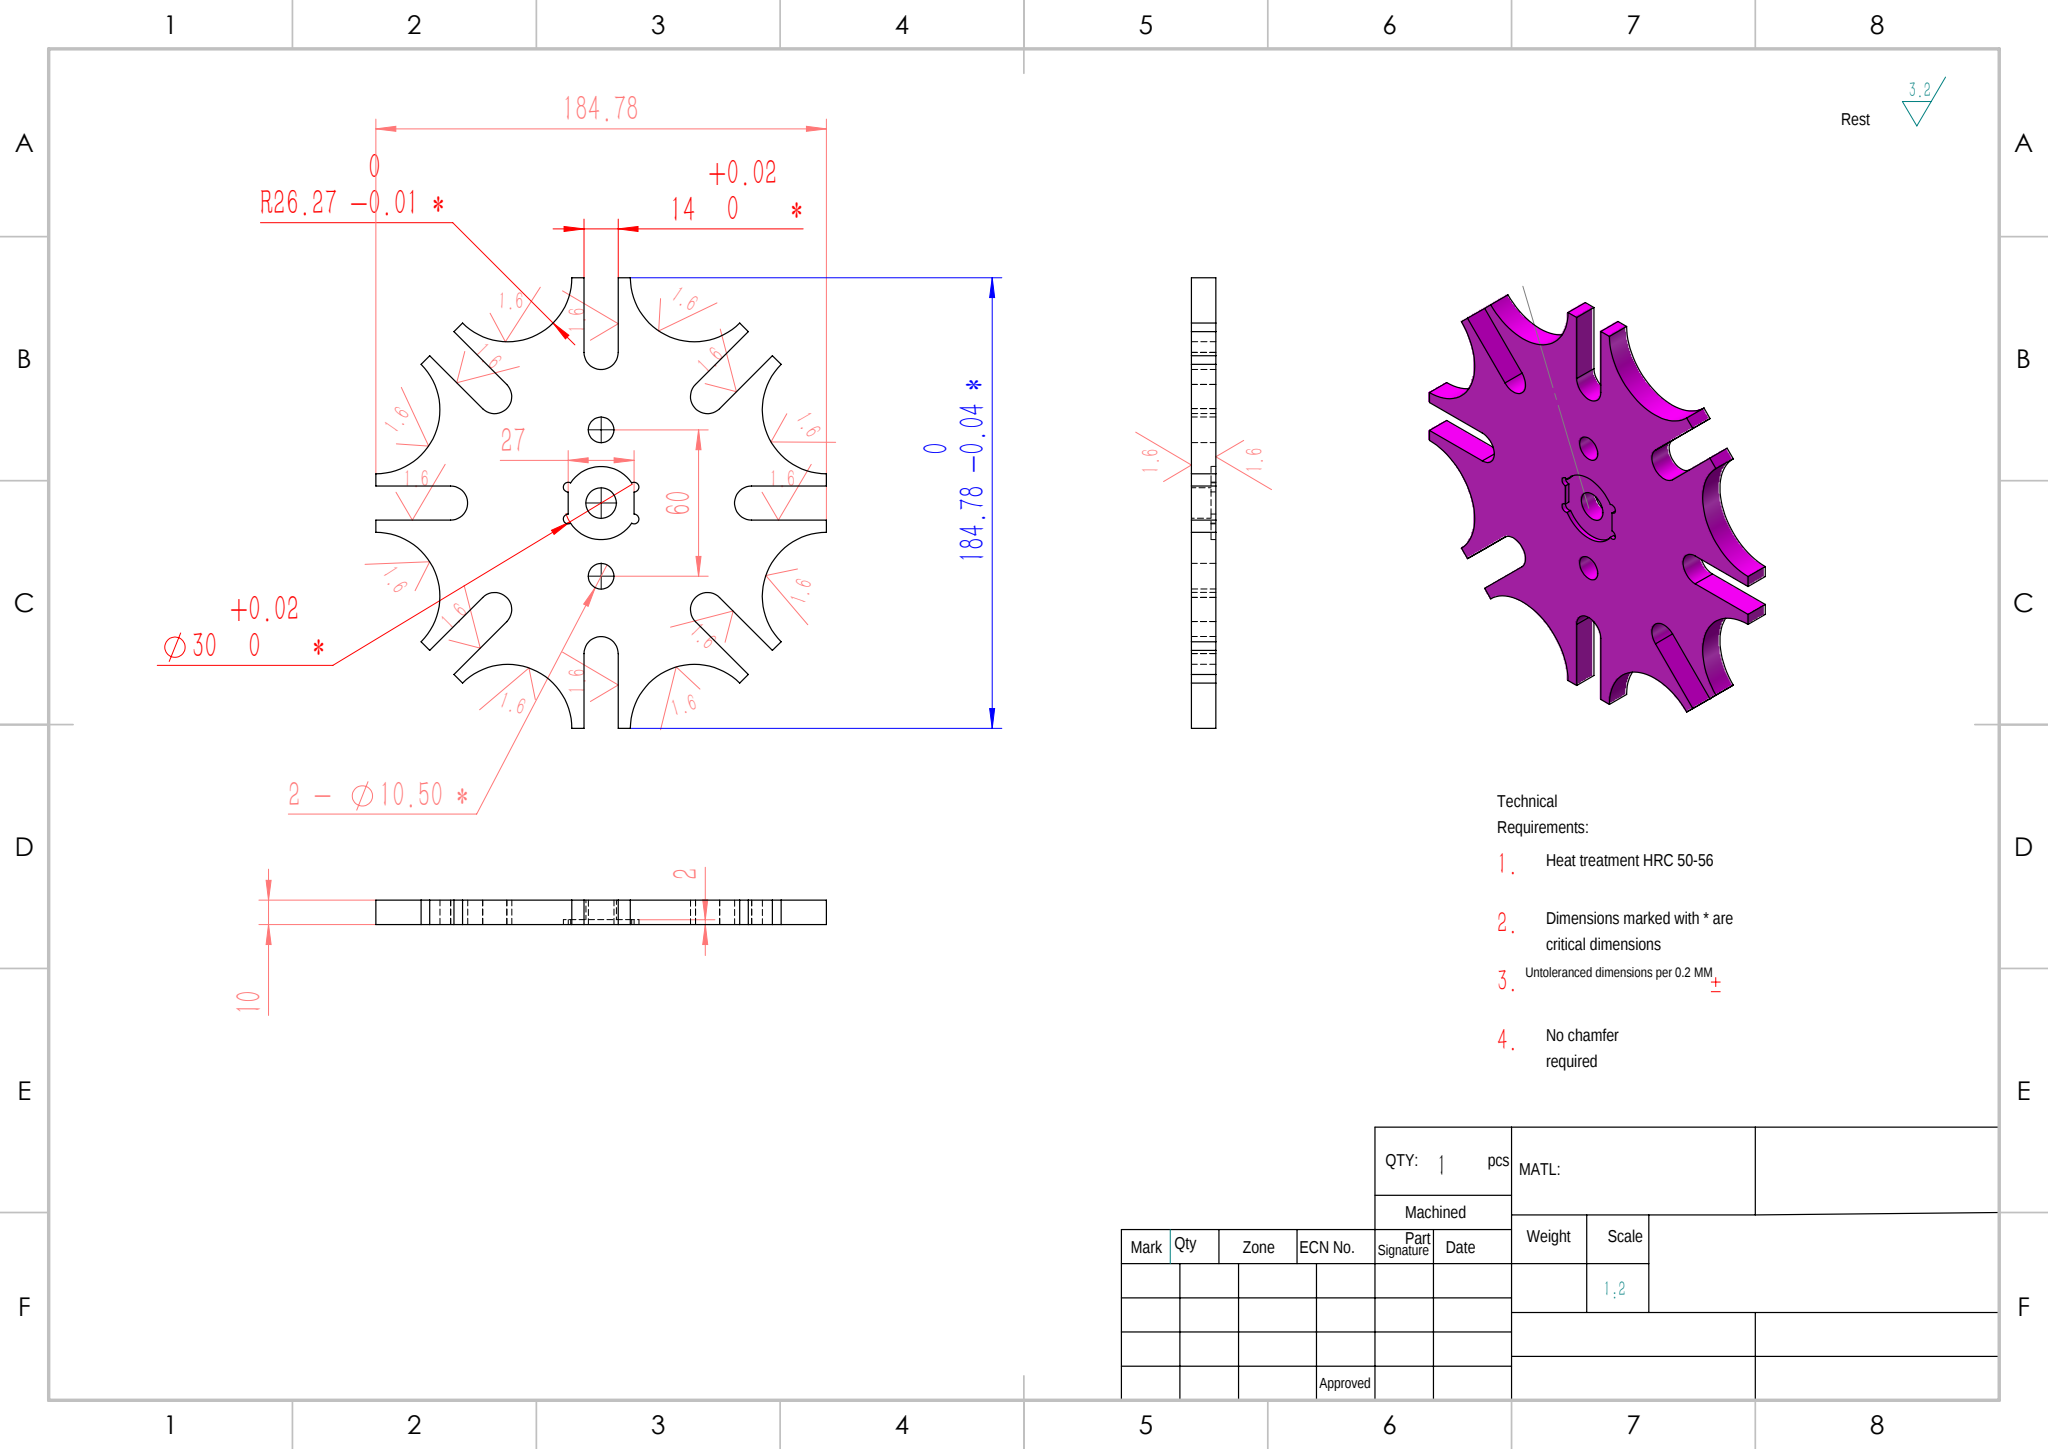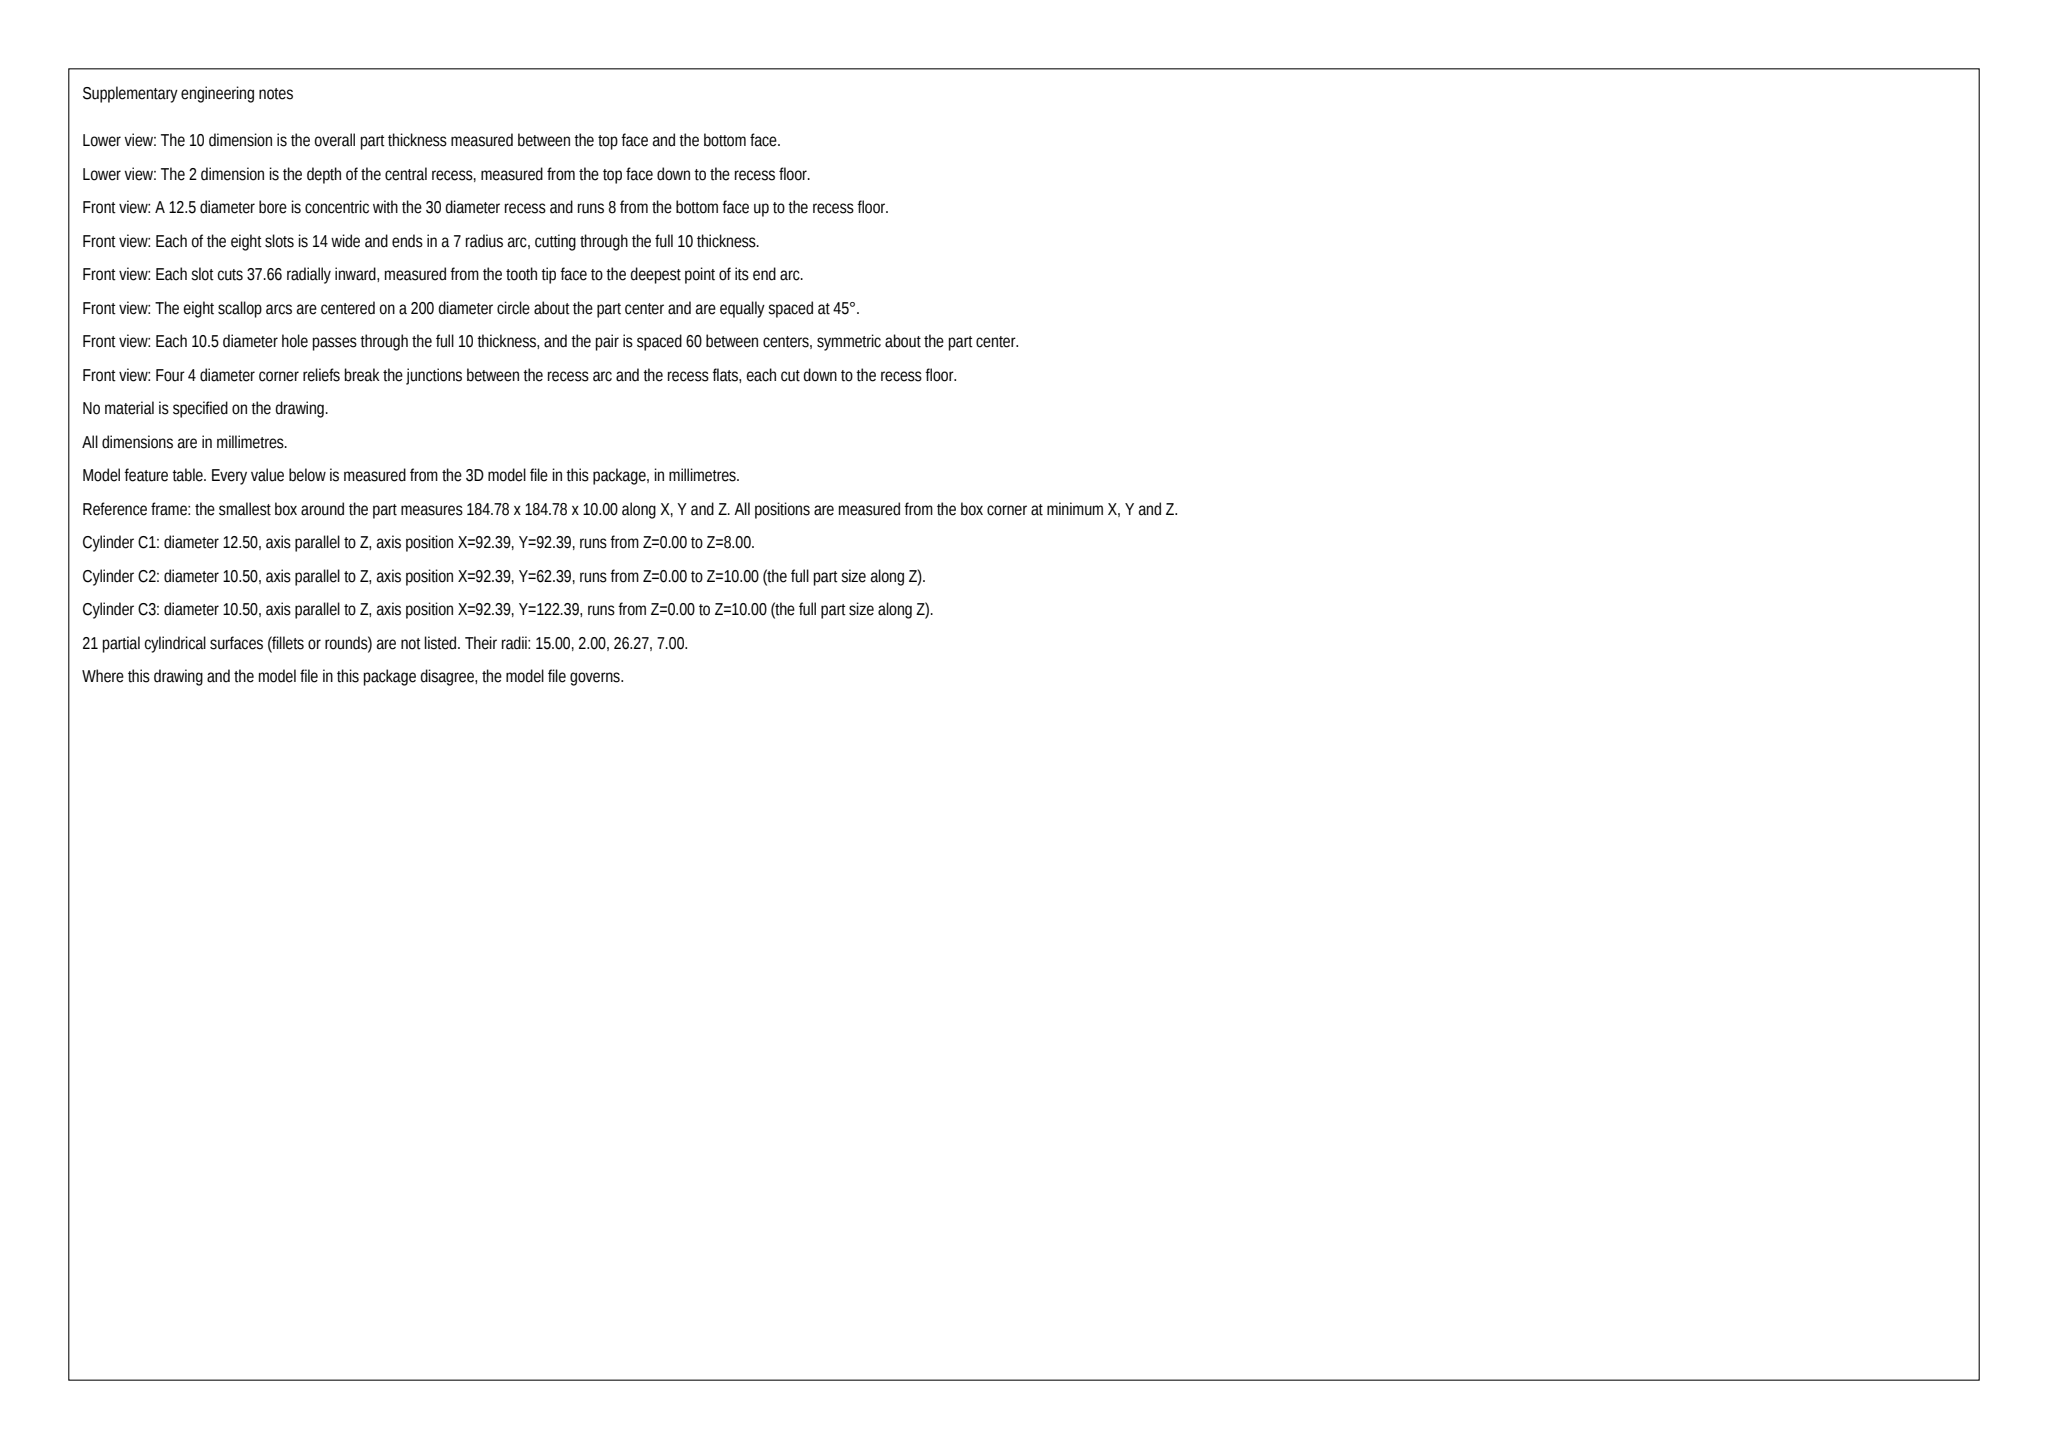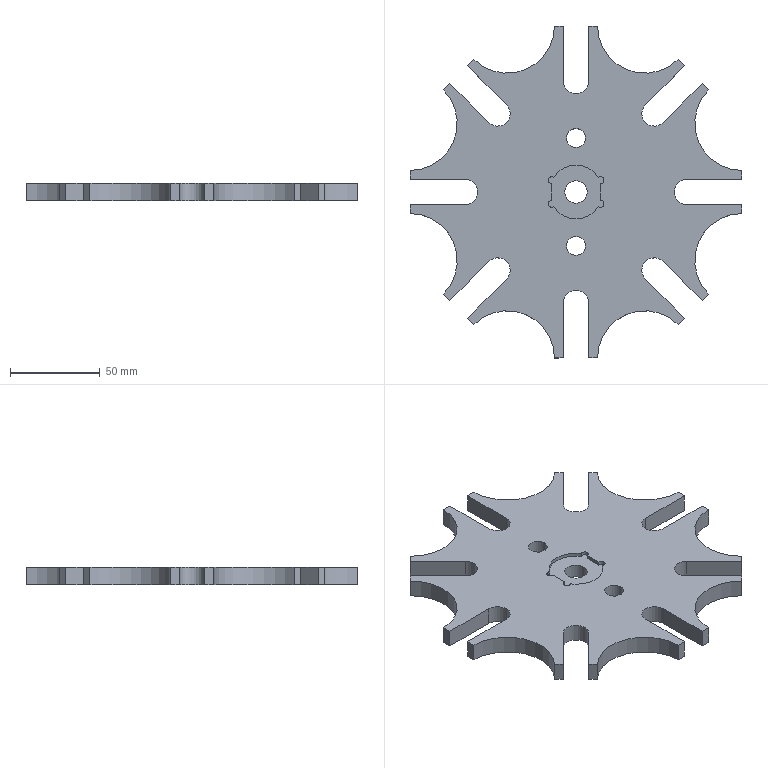Part | SolidWorks | mm | 1 solid | 67 faces | box 184.78 x 184.78 x 10 mm | volume 173184 mm3 | plane 37 | cylinder 30 | commonest cylinder face diameters 52.537 x8 14 x8 4 x6 10.5 x4 12.5 x2 30 x2
Drawing notes:
8X SLOT 14 WIDE: END ARC CTR 61.7 FROM PART CENTER | from the solid: Ø14 slot-end arcs at (154.1,92.4) & (136.0,136.0) vs center (92.4,92.4): 61.7 radial
8X 14 WIDE SLOT, EQ SP 45 DEG ABOUT CENTER | from the solid: 8 off Ø14 180-deg slot-end arcs at 45 deg spacing, radius 61.7
8X R26.27 SCALLOP, CTR 38.3 EA SIDE OF CL ON 184.78 FLATS | from the solid: Ø52.54 arcs at (0,130.7),(0,54.1),(130.7,0),(54.1,0),(184.8,130.7)...; 130.7-92.4=38.3
4X DIAG ARM AT 45: FLANK 30.7 (21.7 X 21.7 PROJ) | from the solid: inclined planes 45/45/90, size 21.7x21.7x10; sqrt(21.7^2+21.7^2)=30.7
DIAG ARM TIP END FACE 4.95 WIDE AT 45 DEG | from the solid: inclined planes 45/45/90 size 3.5x3.5; sqrt(3.5^2+3.5^2)=4.95
DELETE Ø200: MAX ENVELOPE 184.78 ACROSS FLATS | from the solid: bbox_xyz 184.776 x 184.776 x 10.0; no 200 dia feature
BALLOON 44: OUTER SCALLOP R26.27 (WAS Ø200) | from the solid: Ø52.54 concave arcs = R26.27 outer scallops; no Ø200 cylinder exists
HEAT TREAT HRC 50-55; UNSPEC TOL 0.2 MM; NO CHAMFER; * = CRITICAL | from the solid: unscrambled note text; no chamfer/cone faces in STEP (cones list empty)
build123d program:
from build123d import *

# Parameters (mm, degrees)
BOSS_EXTRUDE1_DEPTH = 10
CIRPATTERN1_COUNT   = 8
SKETCH2_R           = 6.25
CUT_EXTRUDE2_DEPTH  = 132.038
CUT_EXTRUDE3_DEPTH  = 2
SKETCH5_R           = 5.25
CUT_EXTRUDE4_DEPTH  = 20
SKETCH6_R           = 2
CUT_EXTRUDE5_DEPTH  = 2


with BuildPart() as part:
    # Sketch1 → Boss-Extrude1 (new body)
    with BuildSketch(Plane.XY):
        with BuildLine():
            Line((-7, 92.388), (-7, 61.732))
            ThreePointArc((-7, 61.732), (-4.95, 56.782), (0, 54.732))
            Line((0, 54.732), (0, 0))
            Line((0, 0), (-38.701, 38.701))
            ThreePointArc((-38.701, 38.701), (-36.651, 43.651), (-38.701, 48.601))
            Line((-38.701, 48.601), (-60.378, 70.278))
            Line((-60.378, 70.278), (-56.843, 73.813))
            ThreePointArc((-56.843, 73.813), (-28.216, 68.119), (-12, 92.388))
            Line((-12, 92.388), (-7, 92.388))
        make_face()
    boss_extrude1 = extrude(amount=BOSS_EXTRUDE1_DEPTH)

    # CirPattern1: Boss-Extrude1 ×8 about axis
    cirpattern1_axis = Axis((0, 0, -0.5), (0, 0, 1))
    for i in range(1, CIRPATTERN1_COUNT):
        add(boss_extrude1.rotate(cirpattern1_axis, i * 360 / CIRPATTERN1_COUNT))

    # Sketch2 → Cut-Extrude2 (cut, through all)
    with BuildSketch(Plane.XY):
        Circle(SKETCH2_R)
    extrude(amount=CUT_EXTRUDE2_DEPTH, mode=Mode.SUBTRACT)

    # Sketch4 → Cut-Extrude3 (cut)
    with BuildSketch(Plane.XY.offset(10)):
        with BuildLine():
            Line((-13.5, 6.538), (-13.5, -6.538))
            ThreePointArc((-13.5, -6.538), (0, -15), (13.5, -6.538))
            Line((13.5, -6.538), (13.5, 6.538))
            ThreePointArc((13.5, 6.538), (0, 15), (-13.5, 6.538))
        make_face()
    extrude(amount=-CUT_EXTRUDE3_DEPTH, mode=Mode.SUBTRACT)

    # Sketch5 → Cut-Extrude4 (cut)
    with BuildSketch(Plane.XY.offset(10)):
        with Locations((0, 30)):
            Circle(SKETCH5_R)
        with Locations((0, -30)):
            Circle(SKETCH5_R)
    extrude(amount=-CUT_EXTRUDE4_DEPTH, mode=Mode.SUBTRACT)

    # Sketch6 → Cut-Extrude5 (cut)
    with BuildSketch(Plane.XY.offset(10)):
        with Locations((-13.5, 6.538)):
            Circle(SKETCH6_R)
        with Locations((-13.5, -6.538)):
            Circle(SKETCH6_R)
        with Locations((13.5, -6.538)):
            Circle(SKETCH6_R)
        with Locations((13.5, 6.538)):
            Circle(SKETCH6_R)
    extrude(amount=-CUT_EXTRUDE5_DEPTH, mode=Mode.SUBTRACT)


solid = part.part